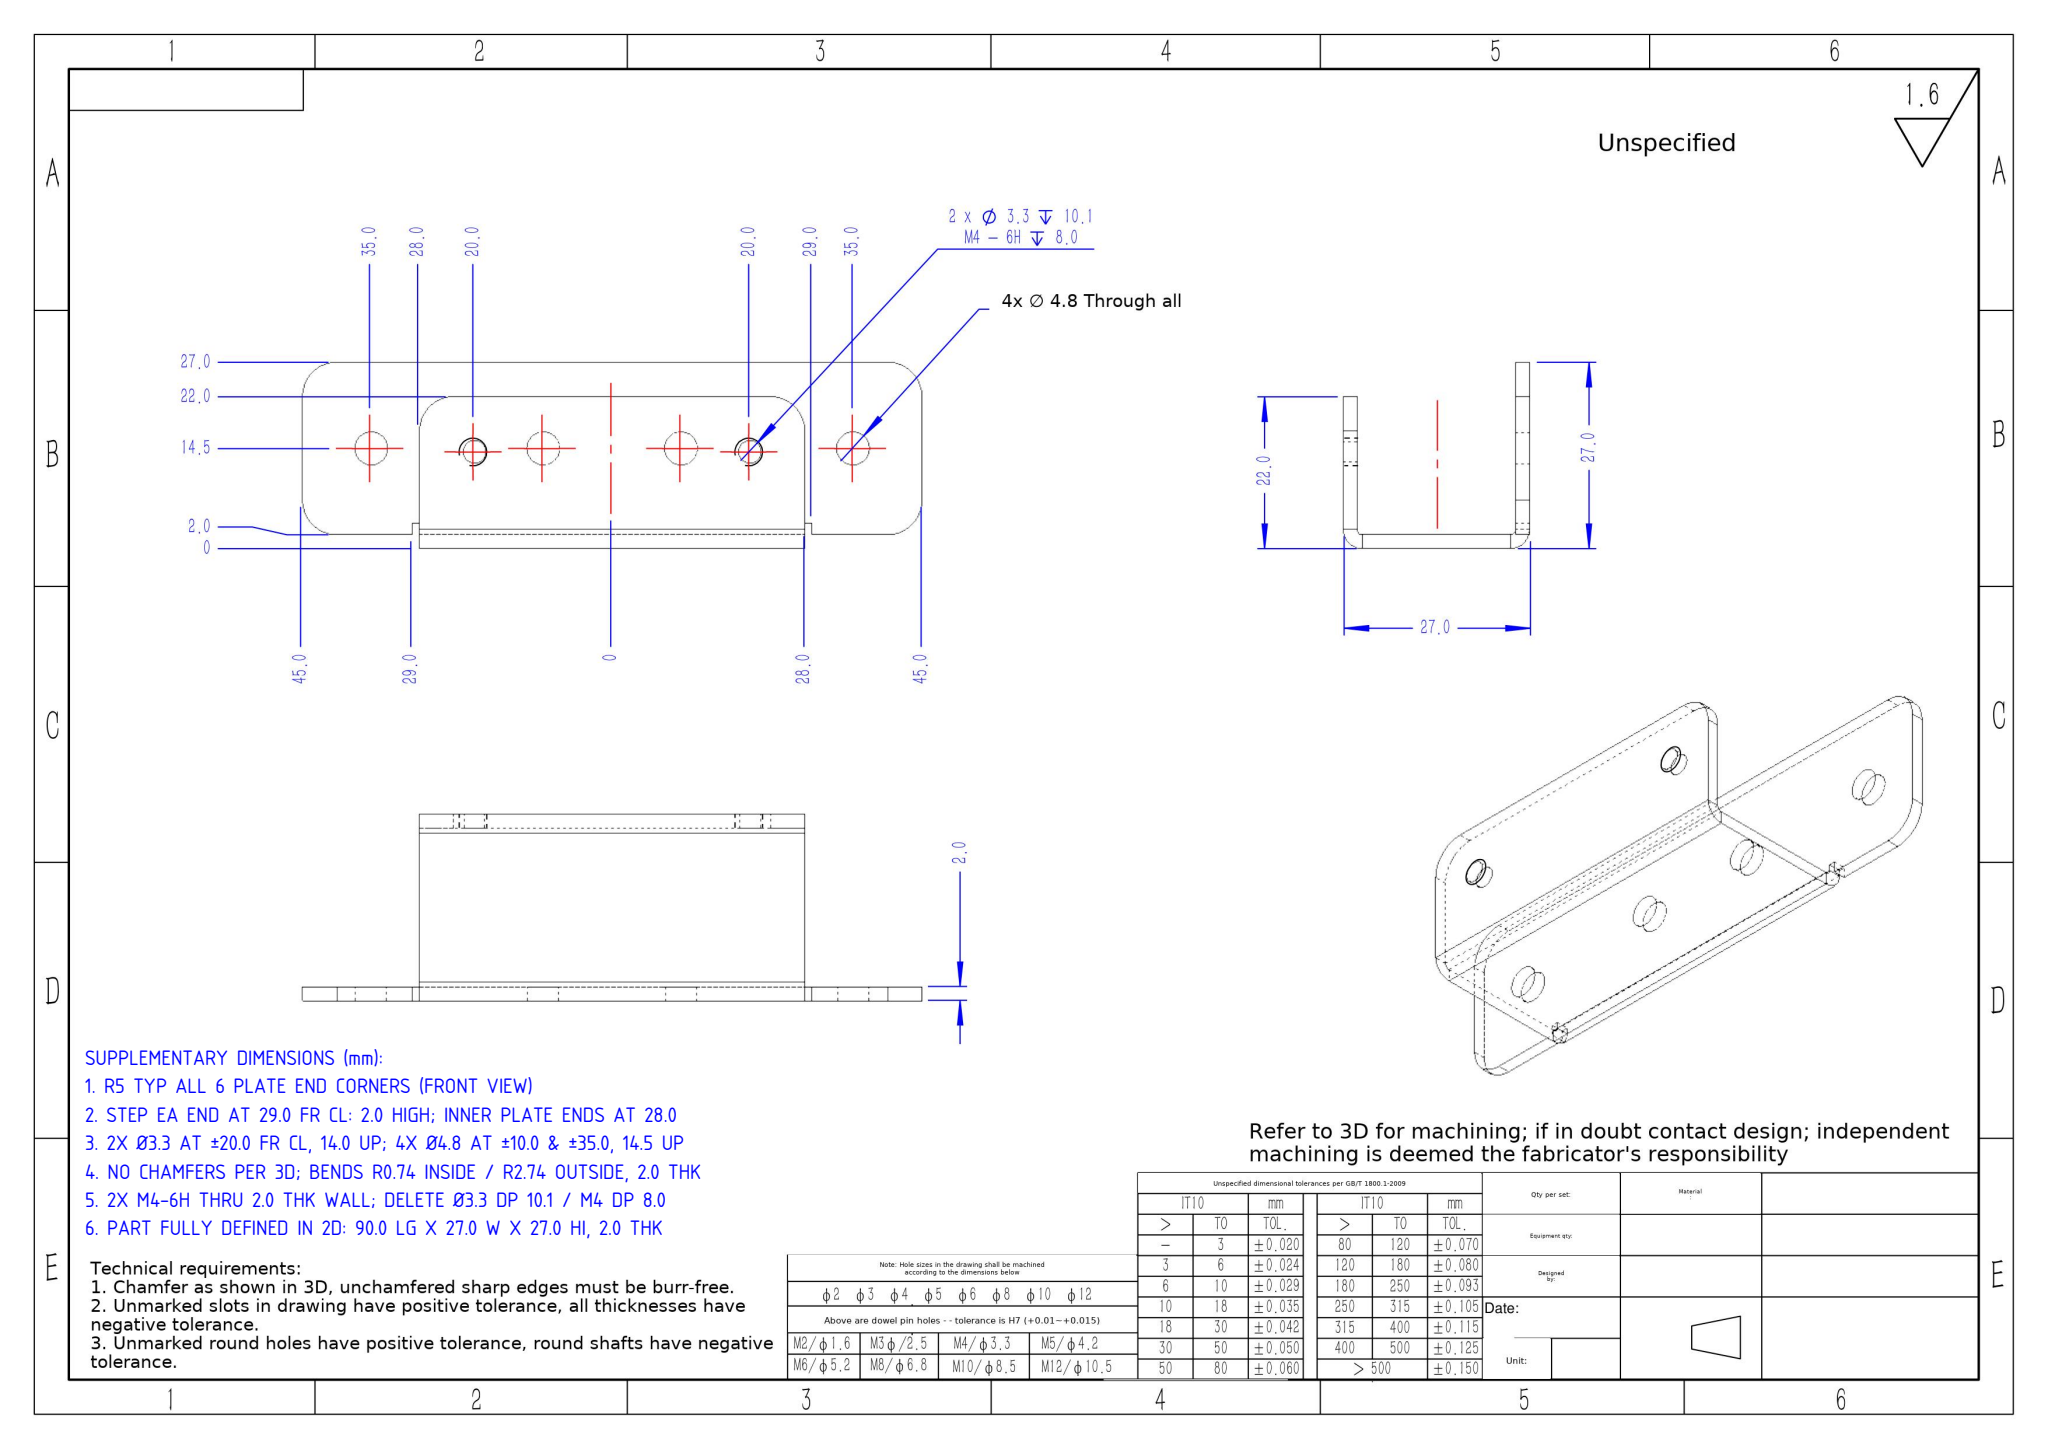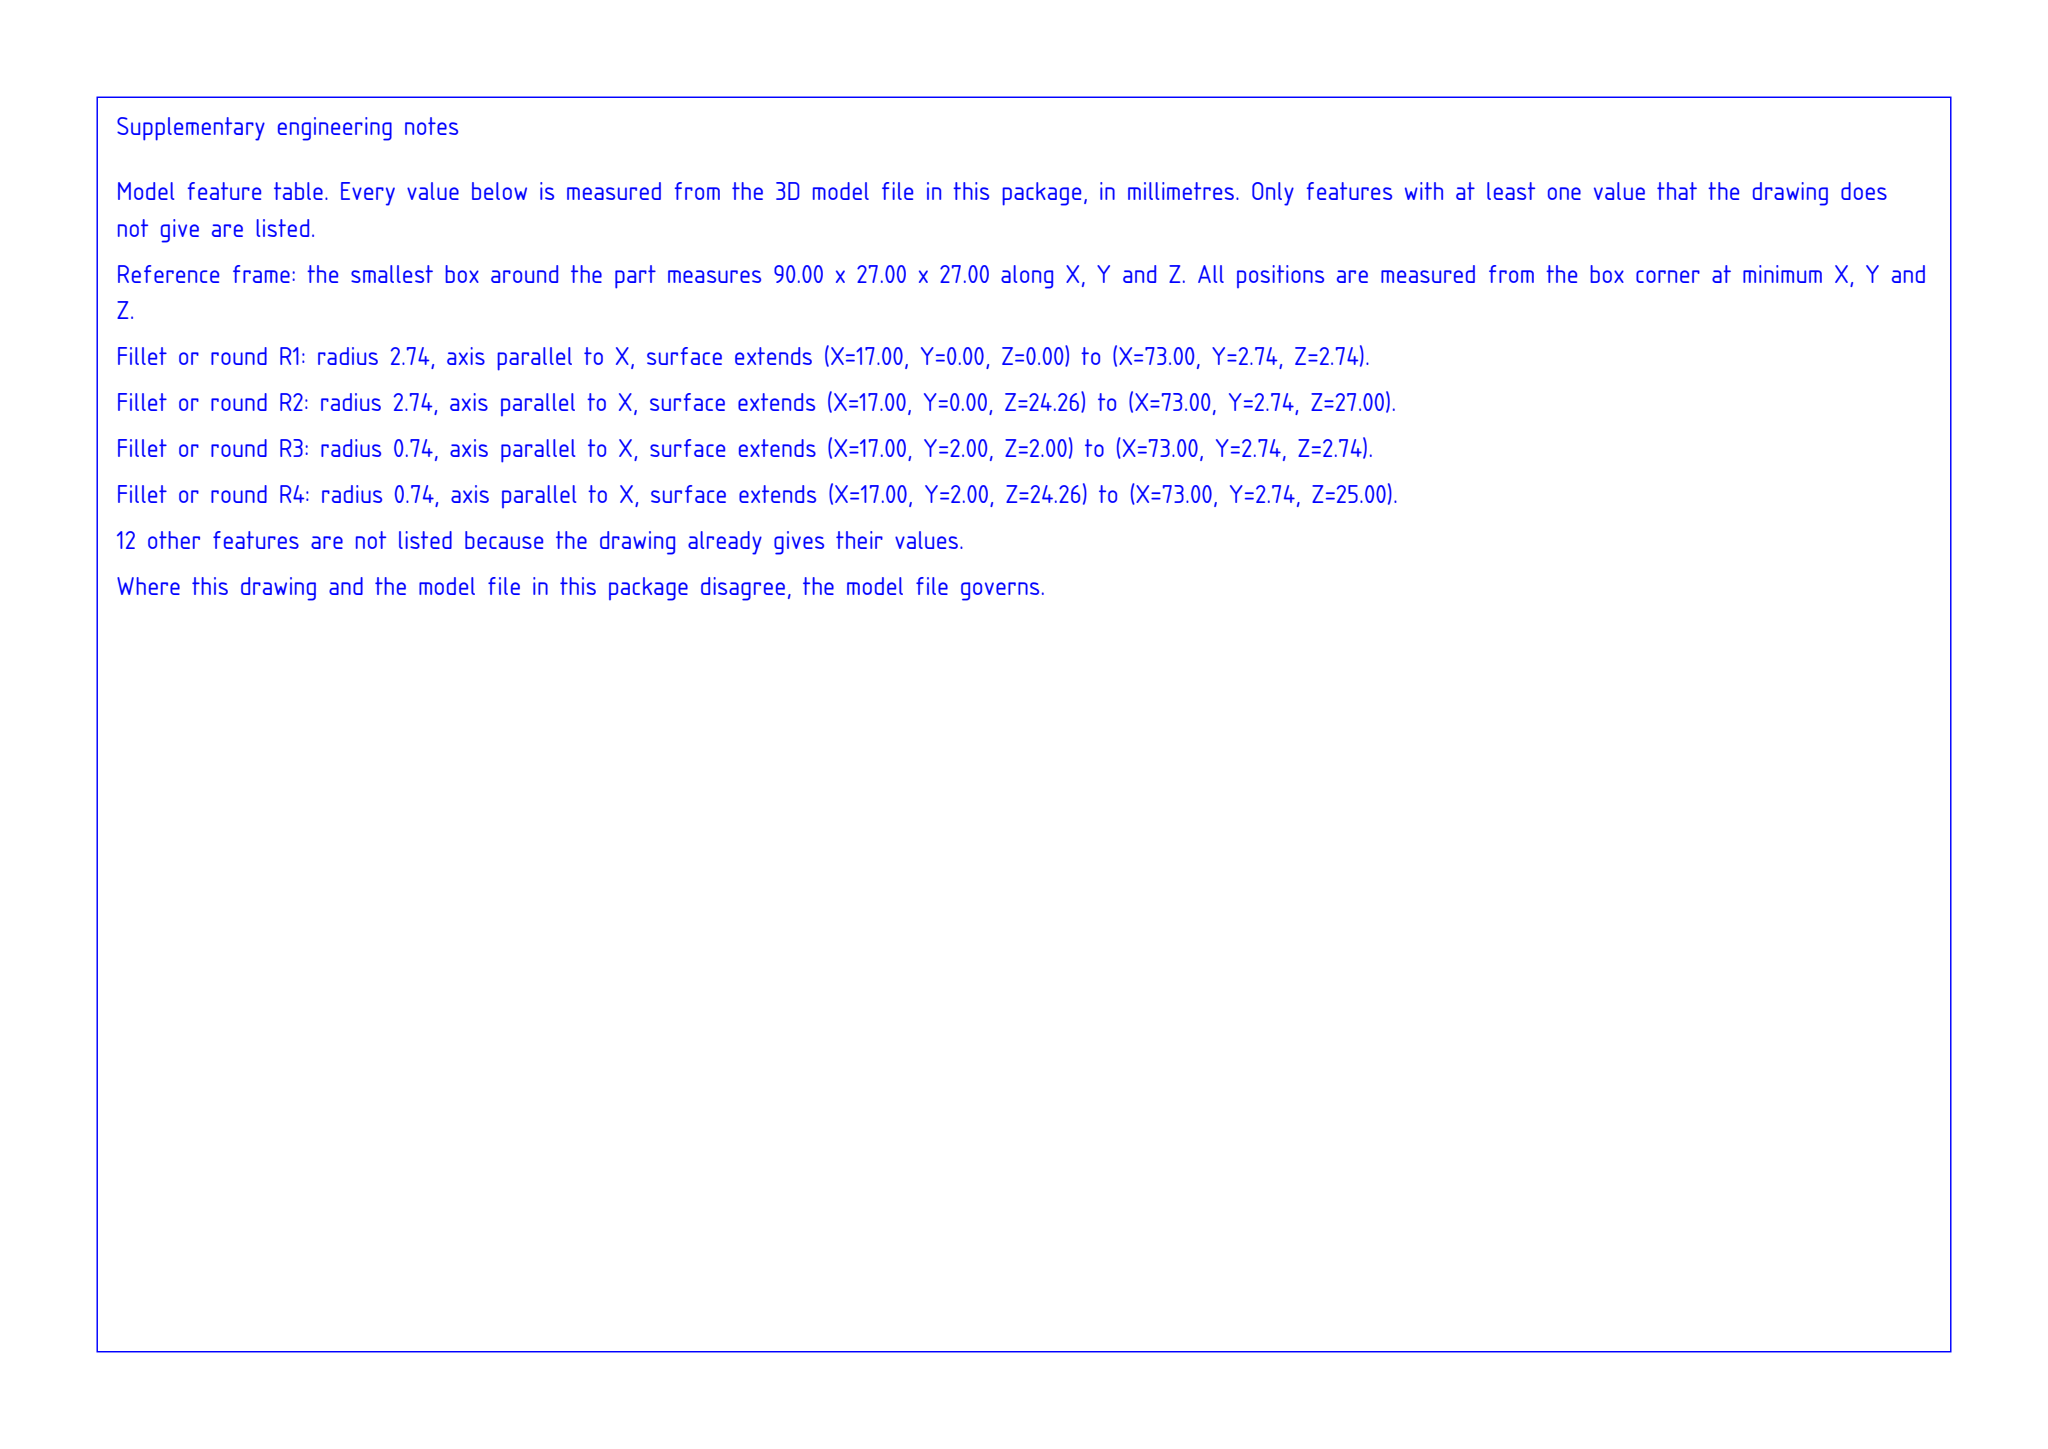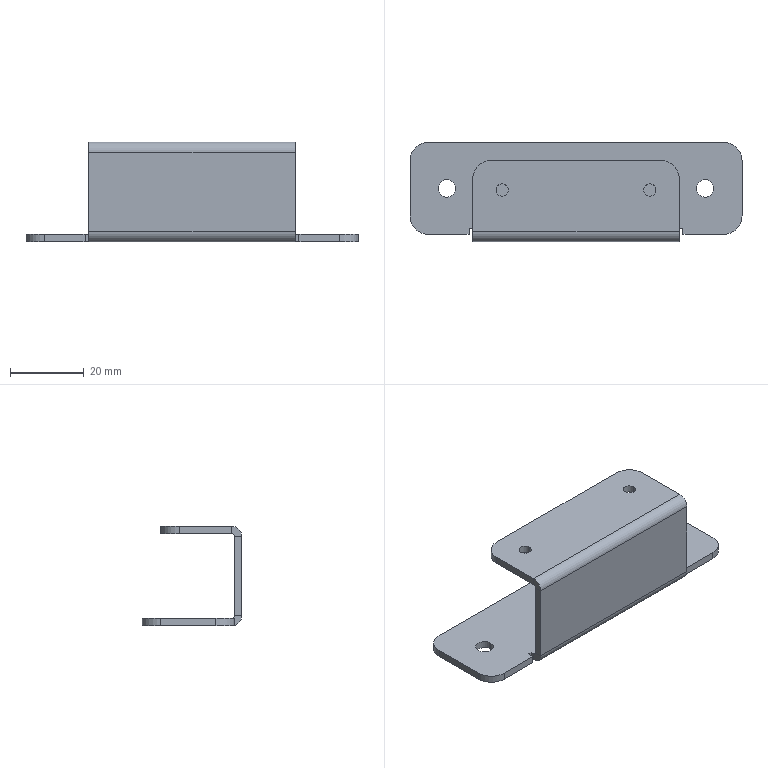Part | SolidWorks | mm | 1 solid | 48 faces | box 90 x 27 x 27 mm | volume 9347 mm3 | plane 26 | cylinder 22 | commonest cylinder face diameters 4.8 x8 10 x6 3.3 x4 5.473 x2 1.473 x2